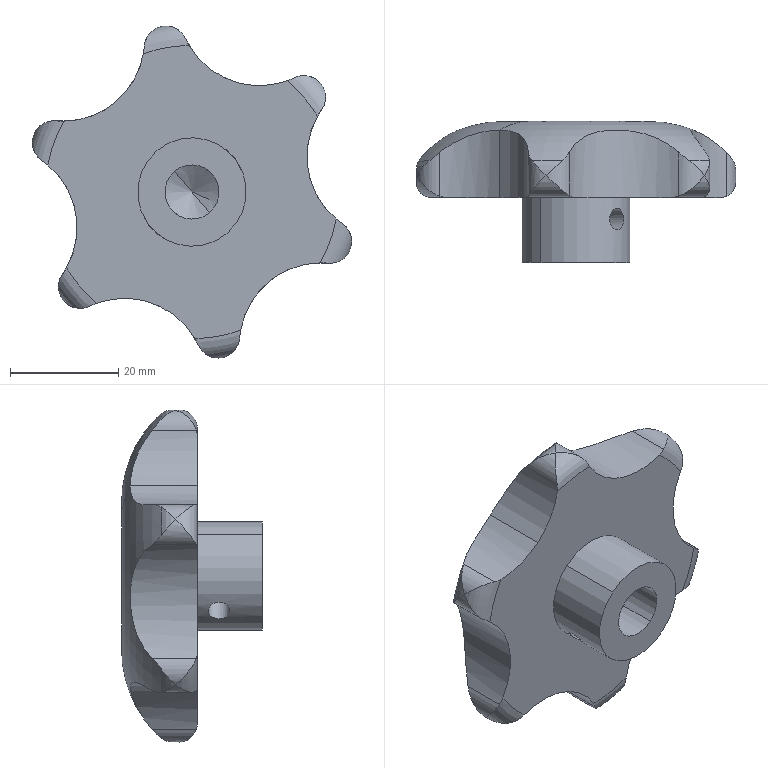Component | SolidWorks | 31-1 | 1 solid | 48 faces | volume 27876 mm3 | cylinder 29 | torus 14 | plane 3 | cone 2 | commonest cylinder face diameters 8 x14 30 x7 4 x4 10 x2 20 x2